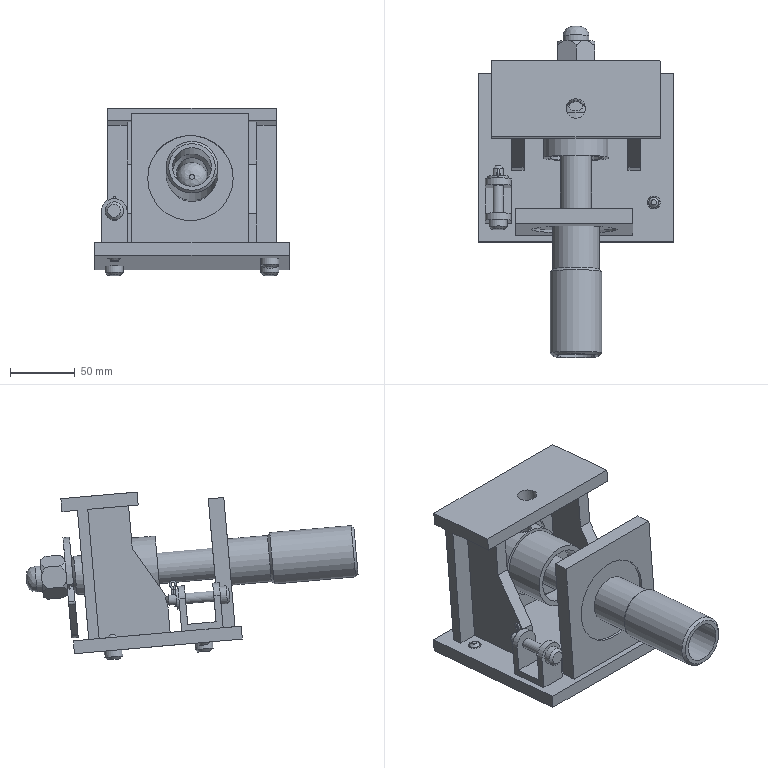Assembly | NX | mm | 14 component files | 14 solids | 166 faces | box 150 x 256.08 x 129.48 mm | volume 770475 mm3 | plane 86 | cylinder 50 | cone 25 | torus 3 | spline 2 | commonest cylinder face diameters 8 x7 20 x6 10 x5 14 x4 30 x3 12 x3 66 x2 1.5 x2
Bill of materials:
unnamed part 1 | 1 |  | U-shaped clevis-style bracket: two parallel flat lugs with rounded tops and aligned through holes, joined by a flat base web, with a short cylindrical stud sticking out below the base.
unnamed part 2 | 1 |  | Thin square flat plate with a central round through hole and a faint concentric circular feature on one face.
unnamed part 3 | 1 |  | Pedestal-style bracket: rectangular base plate with small holes, an upright web with a large central through hole, two angled side gusset ribs, and a top flange plate with a single small hole.
unnamed part 4 | 1 |  | Stepped cylindrical pin with rounded ends, a larger central collar with a radial cross hole, a shoulder step, and a small groove near one end.
unnamed part 5 | 1 |  | Flat, constant-thickness hook- or latch-shaped plate: a rounded head with an open curved notch, tapering to a rounded tail with a small through hole.
unnamed part 6 | 1 |  | Bent round-wire part with a closed eye loop at one end and two parallel straight legs of unequal length, similar in form to a split pin.
unnamed part 7 | 1 |  | Thin-walled cylindrical sleeve with a short larger-diameter collar at one end, and a radial through hole in the collar.
unnamed part 8 | 1 |  | Headed cylindrical pin with a chamfered head, a plain shank, a chamfered tip, and a small cross hole near the tip end.
unnamed part 9 | 1 |  | Stepped hollow tube with two outer diameters, a through bore with an internal step, and a chamfered outer edge at the larger end.
unnamed part 10 | 1 |  | Hexagonal prism body with chamfered corners on both faces and a plain circular through bore, in the shape of a hex nut.
unnamed part 11 | 1 |  | Flat annular ring of uniform thickness with a central round hole, shaped like a plain washer.
unnamed part 12 | 3 |  | Solid stepped pin: a large-diameter cylindrical base with a chamfered bottom edge and a smaller coaxial cylindrical shank with a chamfered tip.
Mates:
1. align lock | hand_nut 1 face | locating_pin 1 face
2. touch align | hand_nut 1 edge | rear_baffle 1 face
3. parallel | rear_baffle 1 face | frame 1 face
4. align lock | nut 1 face | locating_pin 1 face
5. concentric | hook_baffle 1 edge | locating_pin 1 edge
6. touch align | nut 1 edge | hook_baffle 1 face
7. concentric | pin 1 edge | locating_seat 1 edge
8. concentric | base_foot 3 edge | frame 1 edge
9. concentric | small_washer 1 edge | locating_seat 1 edge
10. concentric | base_foot 1 edge | frame 1 edge
11. concentric | base_foot 2 edge | frame 1 edge
12. align lock | sleeve 1 face | locating_pin 1 face